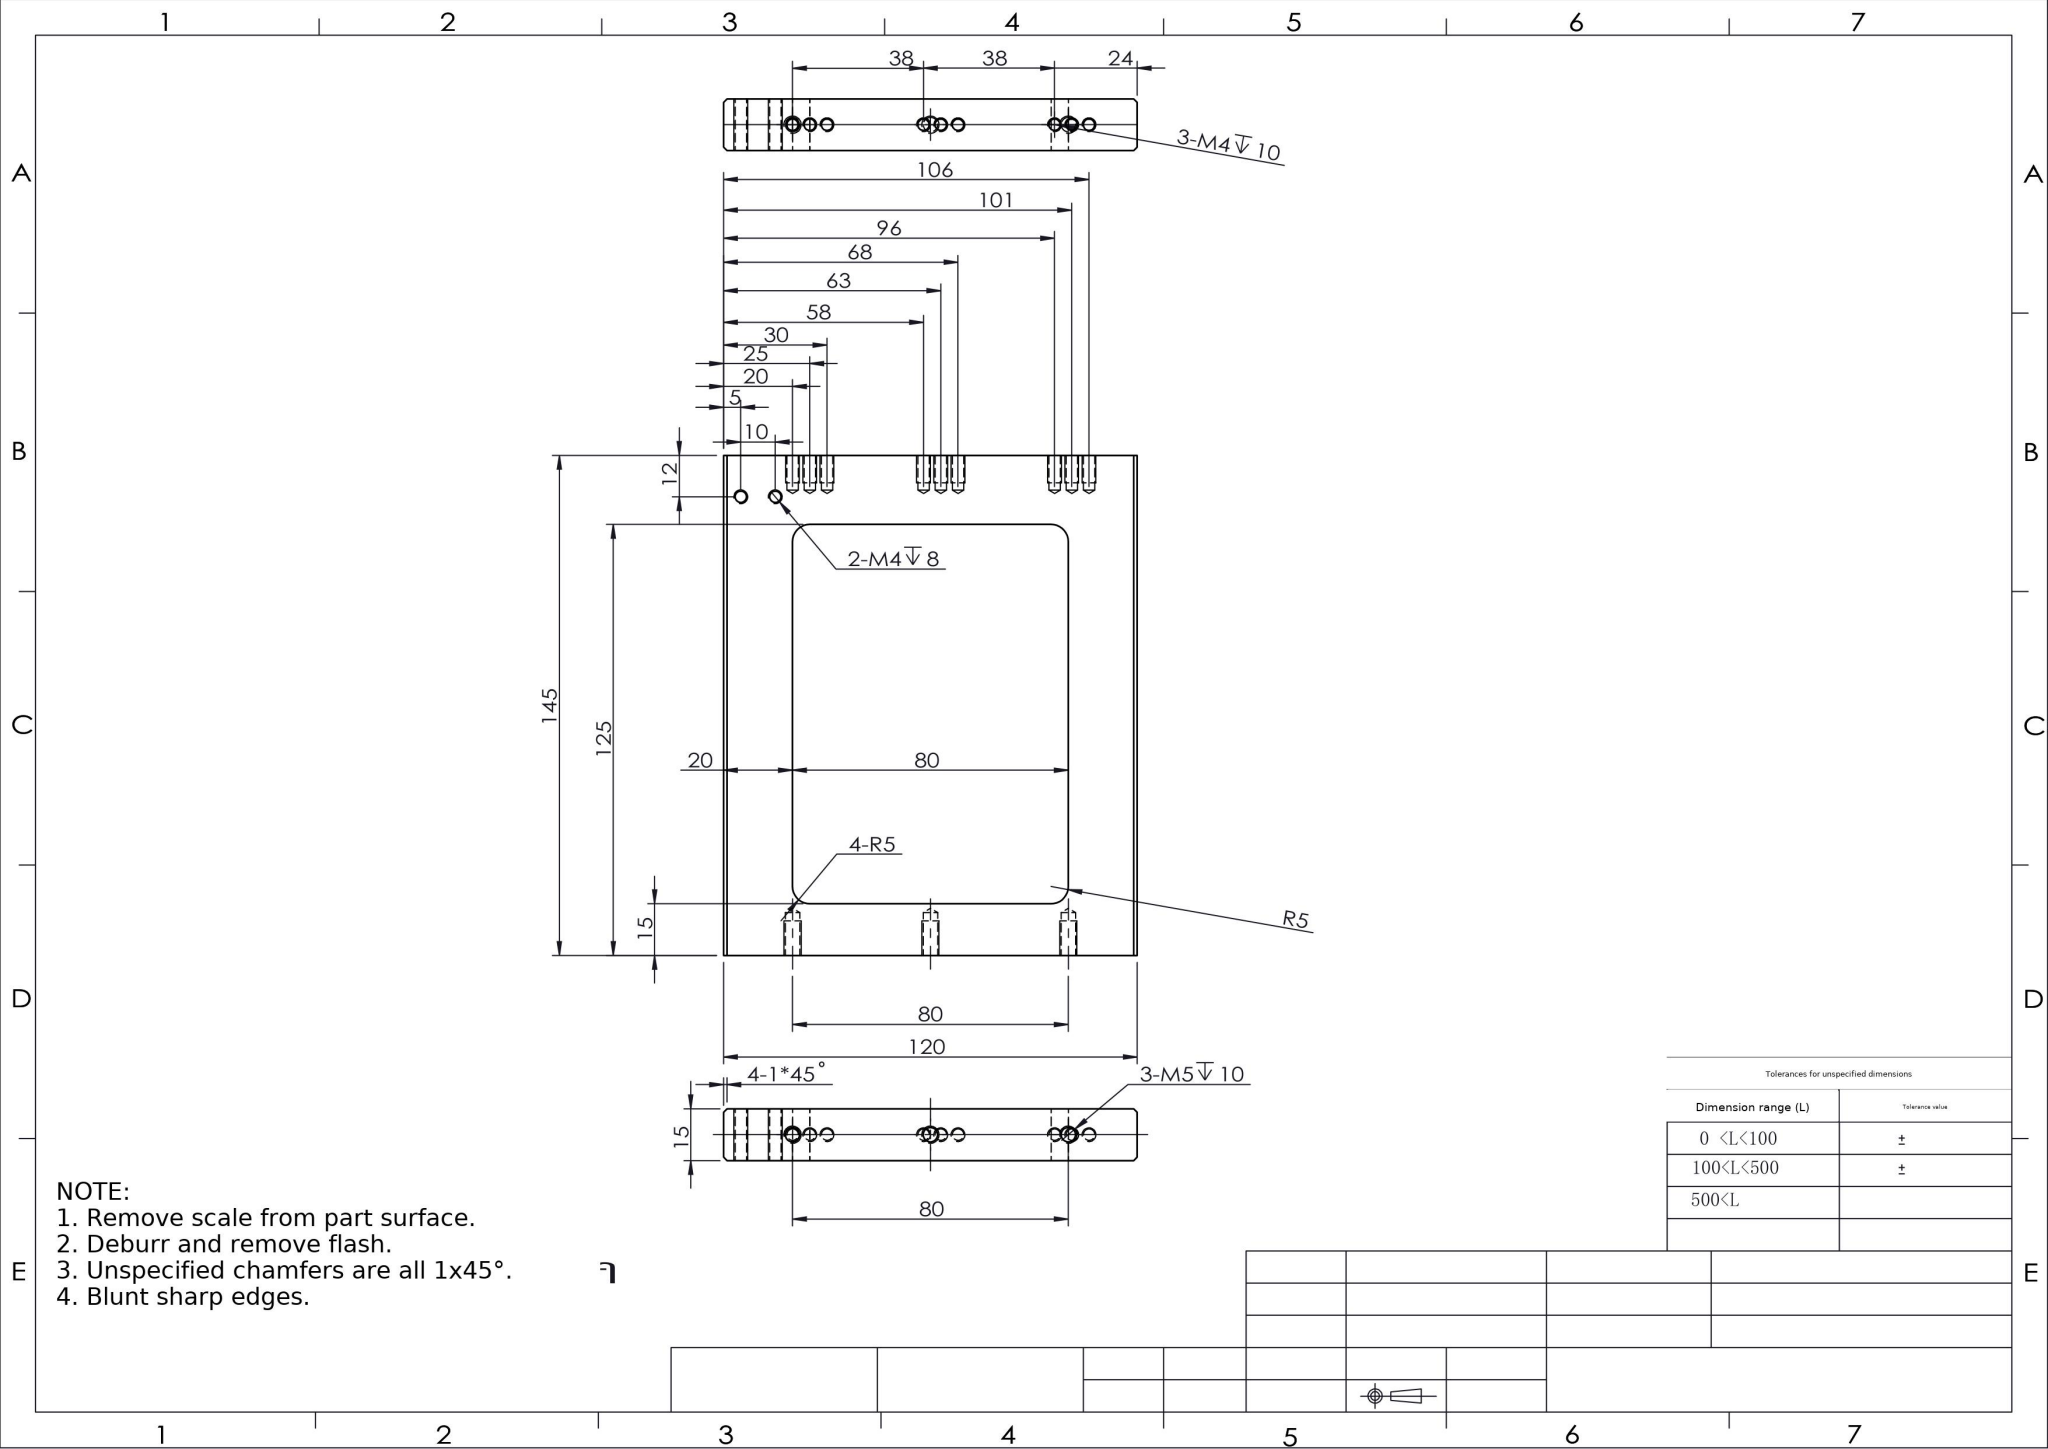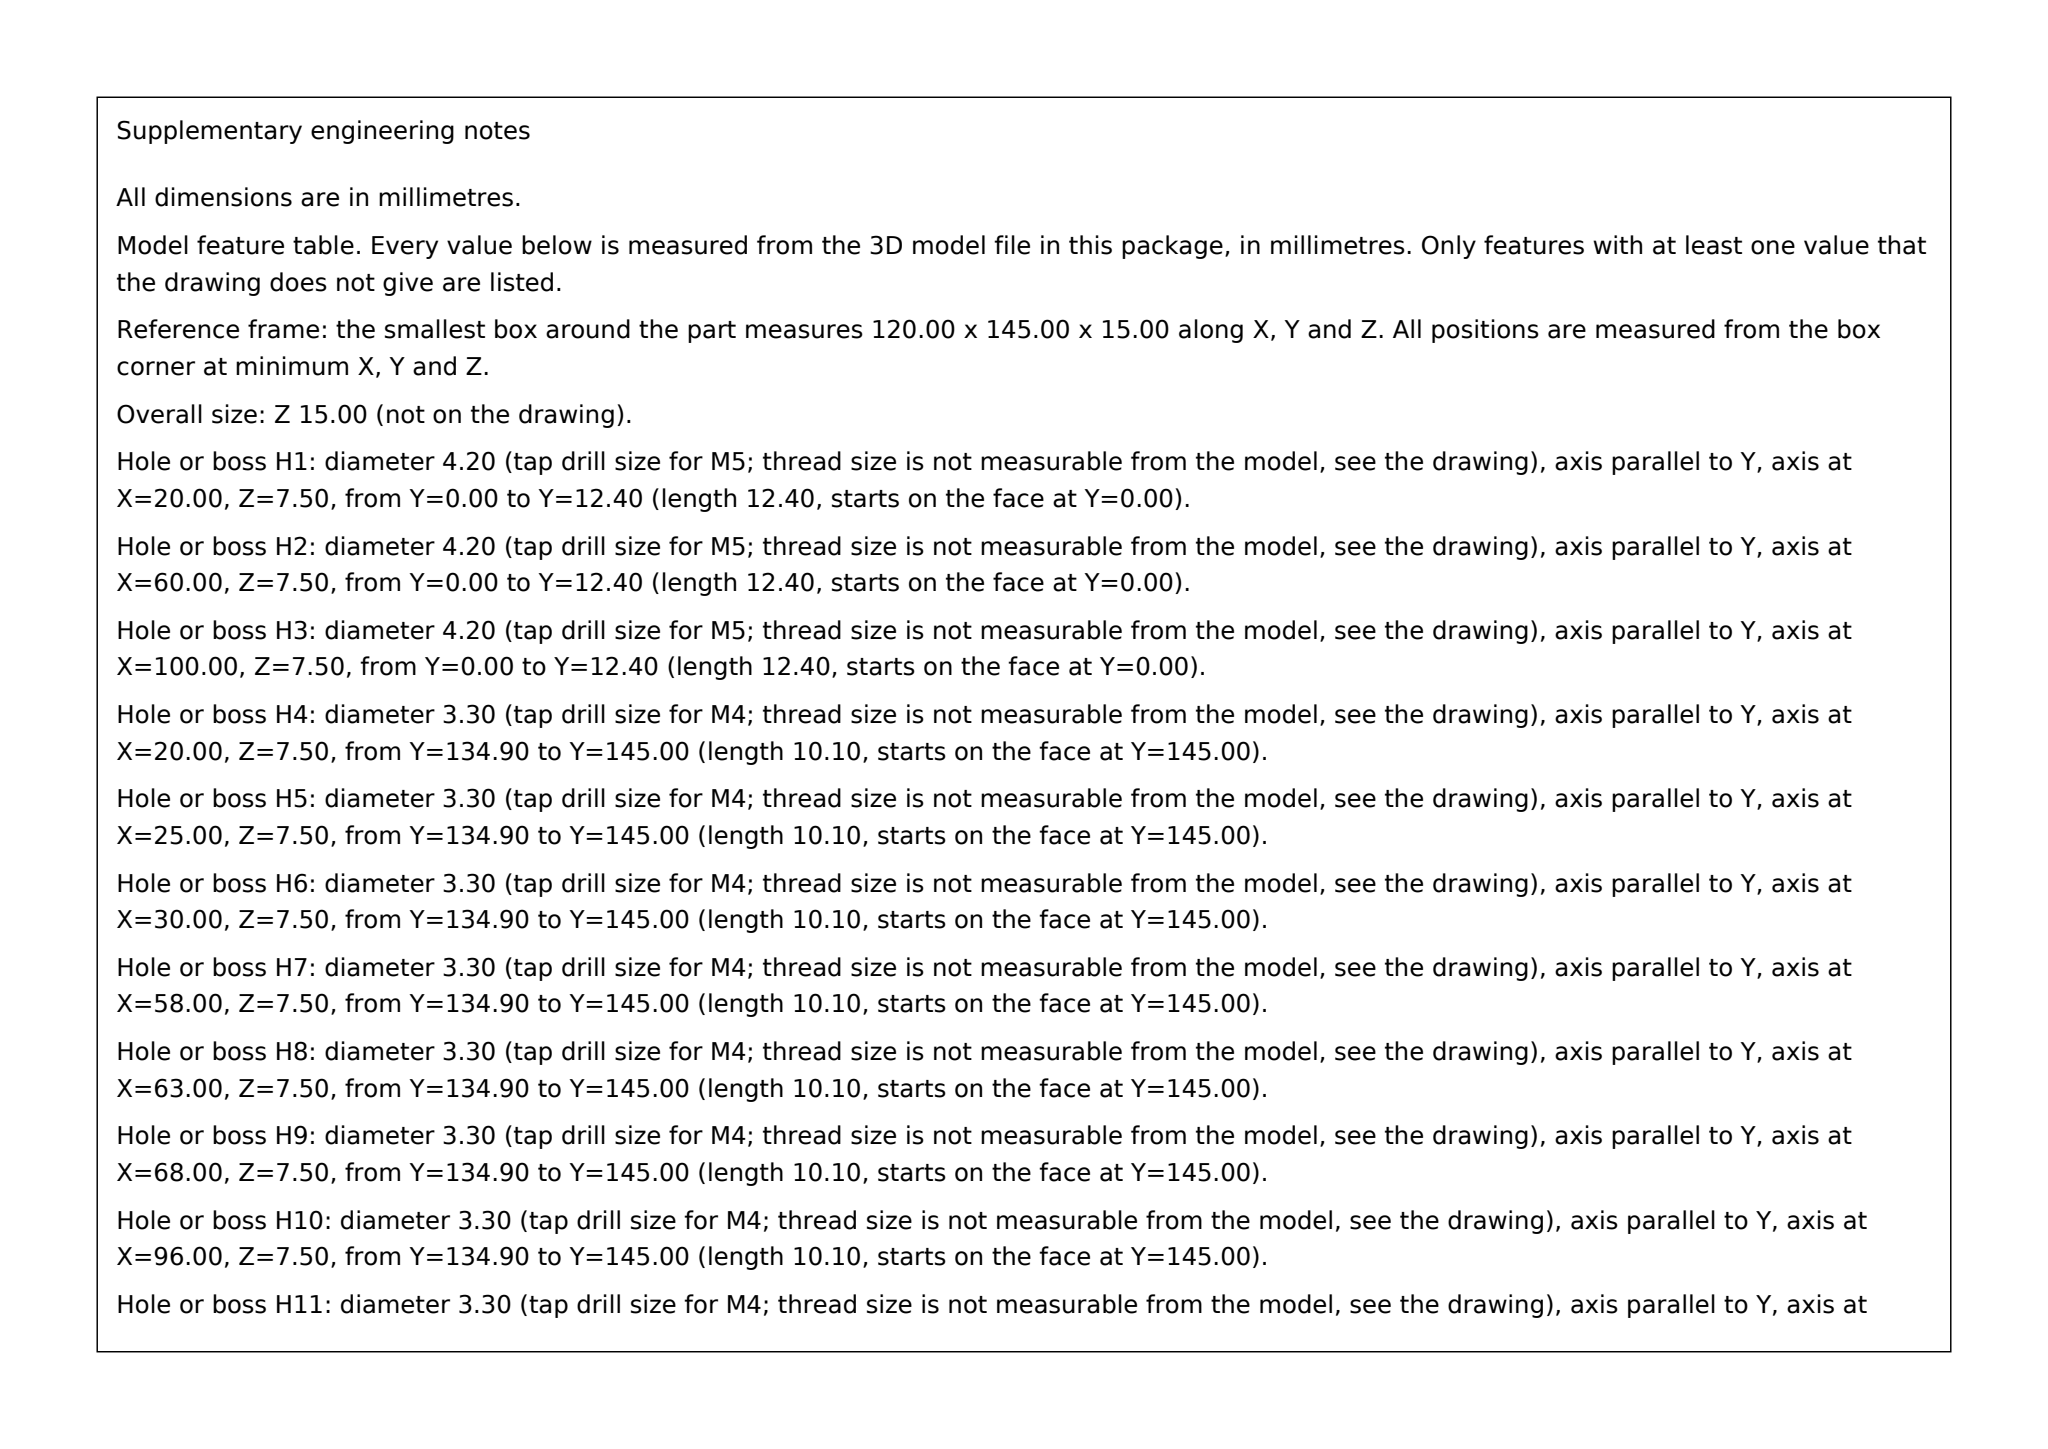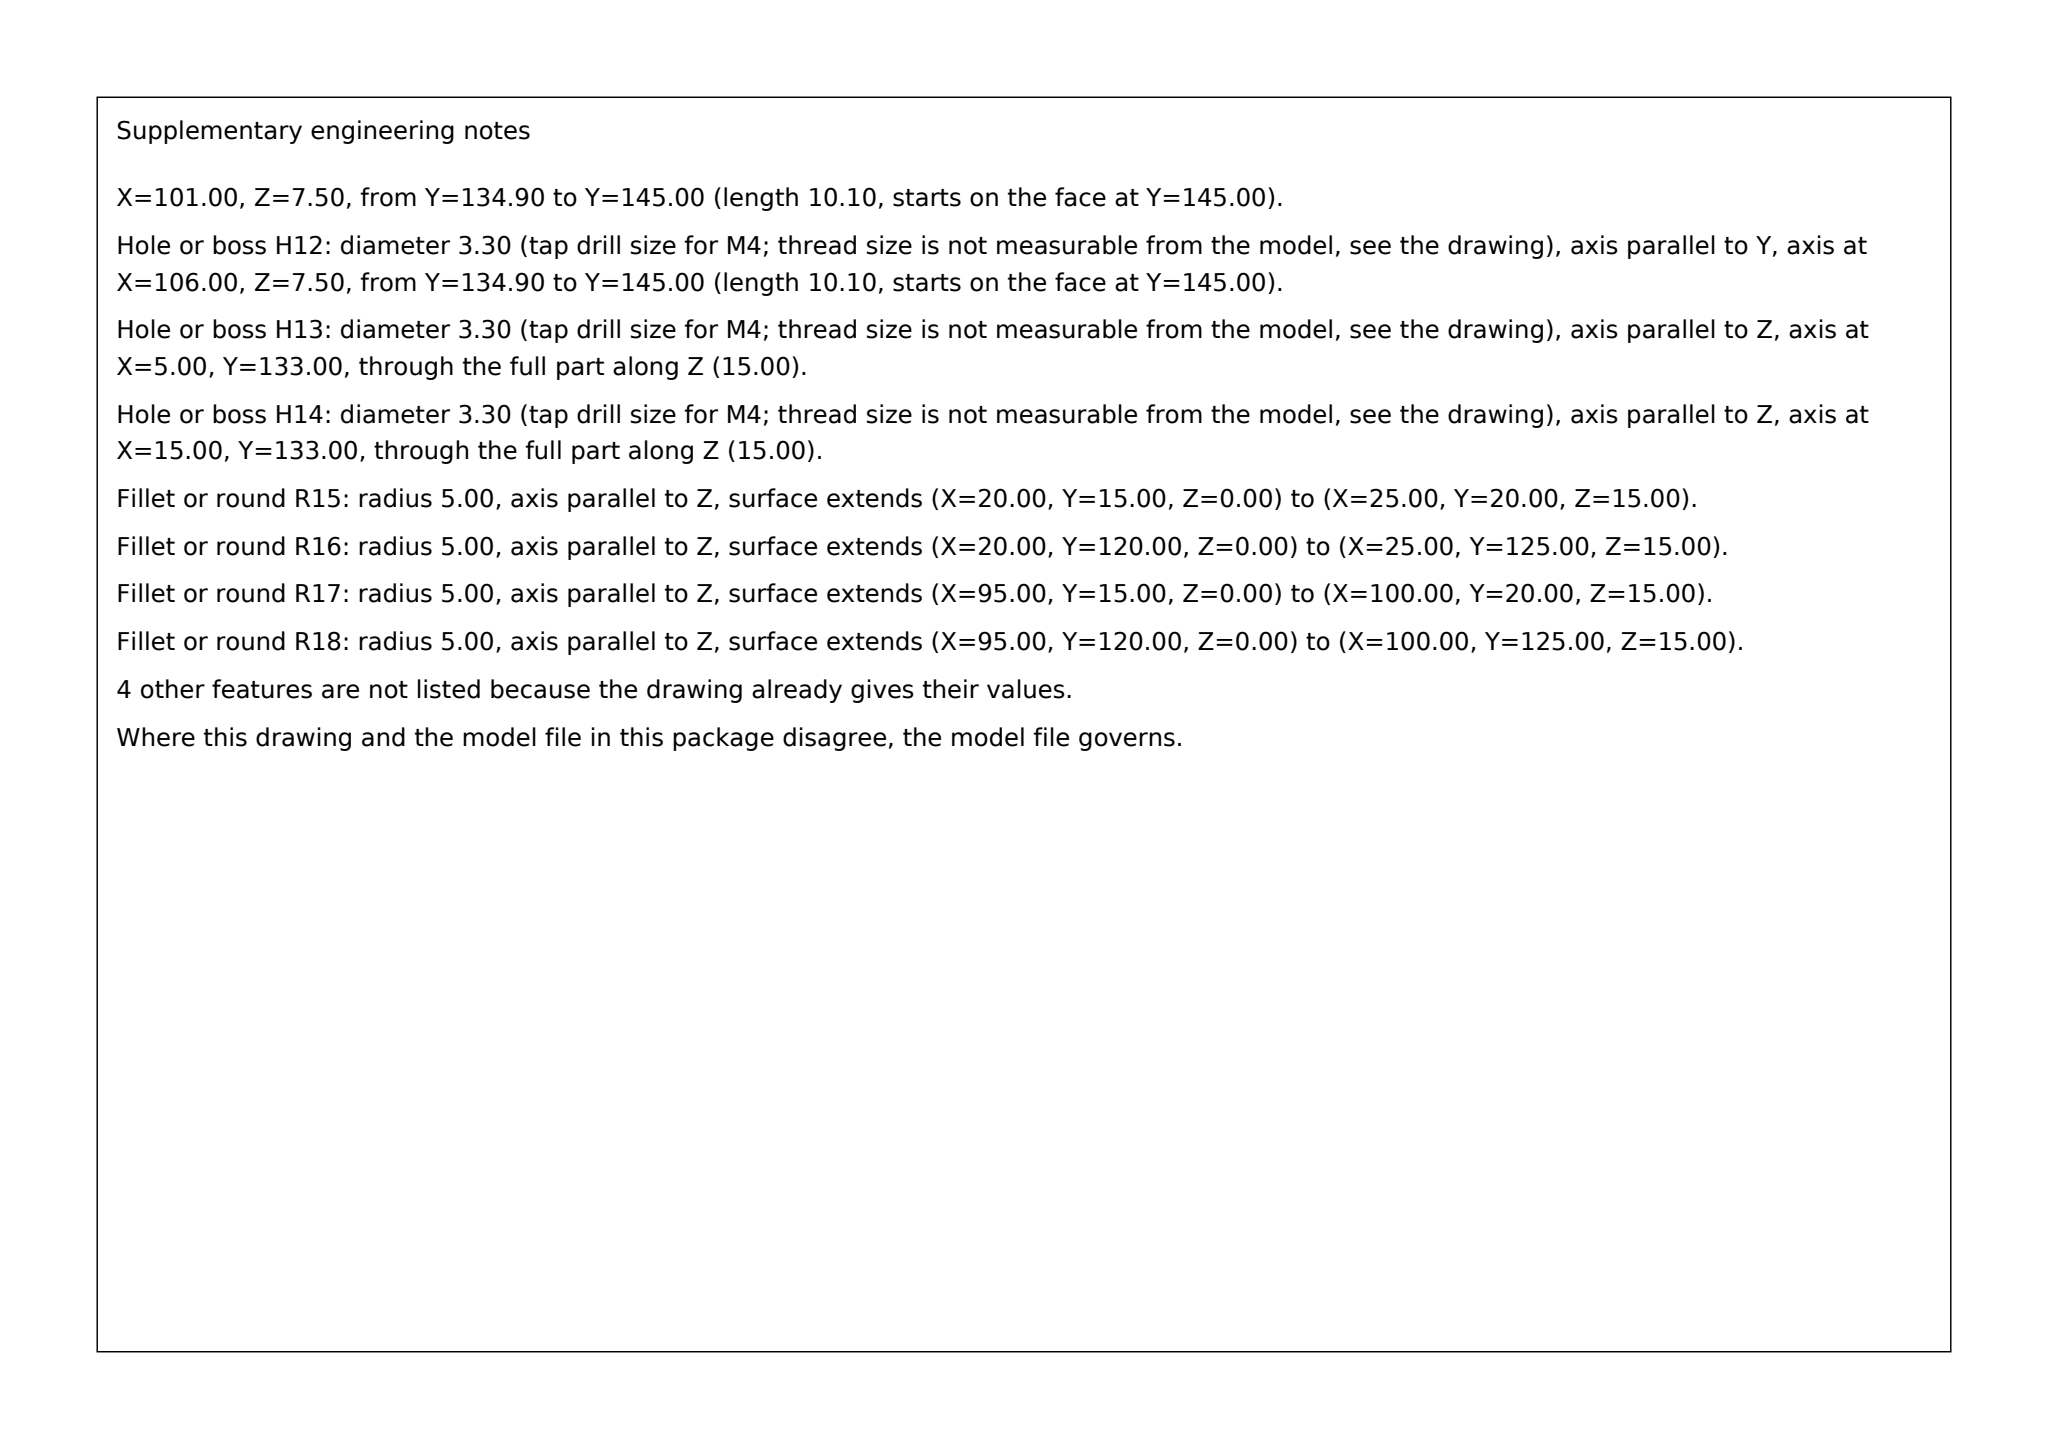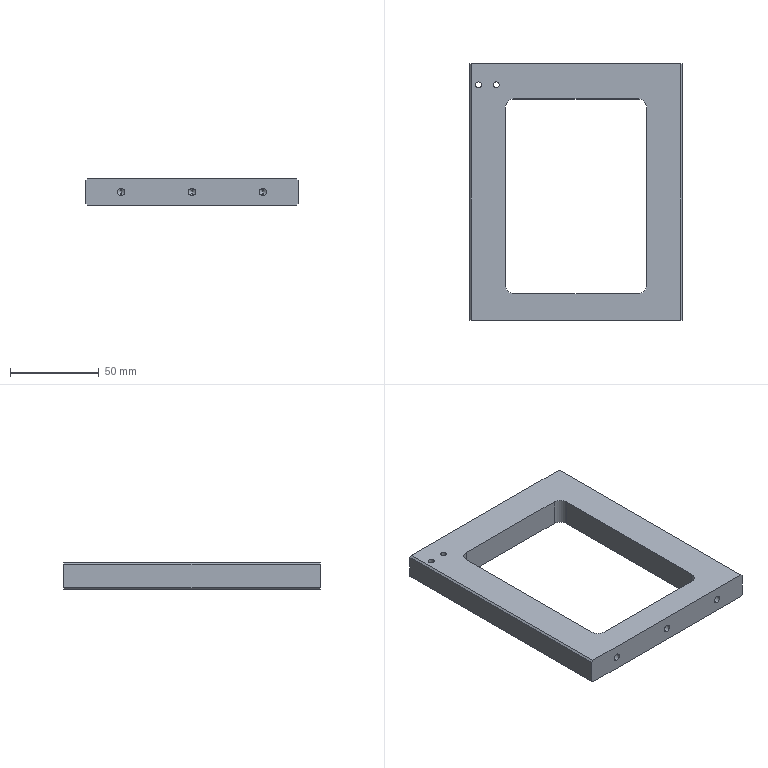Part | SolidWorks | mm | 1 solid | 70 faces | box 120 x 145 x 15 mm | volume 127440 mm3 | cylinder 32 | cone 24 | plane 14 | commonest cylinder face diameters 3.3 x22 4.2 x6 10 x4
build123d program:
from build123d import *

# Parameters (mm, degrees)
SKETCH1_W             = 120
SKETCH1_H             = 145
BOSS_EXTRUDE1_DEPTH   = 15
M5_TAPPED_HOLE1_D     = 4.2
M5_TAPPED_HOLE1_DEPTH = 12.4
M5_TAPPED_HOLE1_TIP   = 1.262
SKETCH7_W             = 80
SKETCH7_H             = 110
CUT_EXTRUDE1_DEPTH    = 189.812
FILLET1_R             = 5
CHAMFER1_SIZE         = 1
SKETCH8_R             = 1.65
CUT_EXTRUDE2_DEPTH    = 189.812
LPATTERN1_COUNT       = 3
LPATTERN1_PITCH       = 38
LPATTERN3_COUNT       = 3
LPATTERN3_PITCH       = 5


with BuildPart() as part:
    # Sketch1 → Boss-Extrude1 (new body)
    with BuildSketch(Plane.XY):
        with Locations((60, 72.5)):
            Rectangle(SKETCH1_W, SKETCH1_H)
    extrude(amount=BOSS_EXTRUDE1_DEPTH)

    # M5 Tapped Hole1
    with Locations(Plane(origin=(0, 0, 0), x_dir=(-1, 0, 0), z_dir=(0, -1, 0))):
        with Locations((-20, -7.5), (-60, -7.5), (-100, -7.5)):
            Hole(M5_TAPPED_HOLE1_D / 2, depth=M5_TAPPED_HOLE1_DEPTH)
            with Locations((0, 0, -(M5_TAPPED_HOLE1_DEPTH + M5_TAPPED_HOLE1_TIP / 2))):  # 118° drill point
                Cone(0, M5_TAPPED_HOLE1_D / 2, M5_TAPPED_HOLE1_TIP, mode=Mode.SUBTRACT)

    # Sketch7 → Cut-Extrude1 (cut, through all)
    with BuildSketch(Plane.XY.offset(15)):
        with Locations((60, 70)):
            Rectangle(SKETCH7_W, SKETCH7_H)
    extrude(amount=-CUT_EXTRUDE1_DEPTH, mode=Mode.SUBTRACT)

    # Fillet1
    fillet1_edges = [part.edges().sort_by_distance(p)[0] for p in [
        (20, 15, 7.5),
        (20, 125, 7.5),
        (100, 125, 7.5),
        (100, 15, 7.5),
    ]]
    fillet(fillet1_edges, radius=FILLET1_R)

    # Chamfer1
    chamfer1_edges = [part.edges().sort_by_distance(p)[0] for p in [
        (120, 72.5, 15),
        (0, 72.5, 15),
        (120, 72.5, 0),
        (0, 72.5, 0),
    ]]
    chamfer(chamfer1_edges, length=CHAMFER1_SIZE)

    # Sketch8 → Cut-Extrude2 (cut, through all)
    with BuildSketch(Plane(origin=(0, 0, 0), x_dir=(-1, 0, 0), z_dir=(0, 0, -1))):
        with Locations((-15, 133)):
            Circle(SKETCH8_R)
        with Locations((-5, 133)):
            Circle(SKETCH8_R)
    extrude(amount=-CUT_EXTRUDE2_DEPTH, mode=Mode.SUBTRACT)

    # Sketch4 → M4 Tapped Hole1 (revolve, cut)
    with BuildSketch(Plane(origin=(20, 145, 7.5), x_dir=(0, 0, 1), z_dir=(1, 0, 0))):
        Polygon((0, 0), (0, 11.091), (1.65, 10.1), (1.65, 0), align=None)
    m4_tapped_hole1 = revolve(axis=Axis((20, 151.35, 7.5), (0, -1, 0)), mode=Mode.SUBTRACT)

    # LPattern1: M4 Tapped Hole1 ×3
    with Locations(*[(i * LPATTERN1_PITCH, 0, 0) for i in range(1, LPATTERN1_COUNT)]):
        add(m4_tapped_hole1, mode=Mode.SUBTRACT)

    # LPattern3: M4 Tapped Hole1 ×3
    with Locations(*[(i * LPATTERN3_PITCH, 0, 0) for i in range(1, LPATTERN3_COUNT)]):
        add(m4_tapped_hole1, mode=Mode.SUBTRACT)

    # LPattern3 copy 1 sketch → LPattern3 copy 1 (revolve, cut)
    with BuildSketch(Plane(origin=(63, 145, 7.5), x_dir=(0, 0, 1), z_dir=(1, 0, 0))):
        Polygon((0, 0), (0, 11.091), (1.65, 10.1), (1.65, 0), align=None)
    revolve(axis=Axis((63, 151.35, 7.5), (0, -1, 0)), mode=Mode.SUBTRACT)

    # LPattern3 copy 2 sketch → LPattern3 copy 2 (revolve, cut)
    with BuildSketch(Plane(origin=(68, 145, 7.5), x_dir=(0, 0, 1), z_dir=(1, 0, 0))):
        Polygon((0, 0), (0, 11.091), (1.65, 10.1), (1.65, 0), align=None)
    revolve(axis=Axis((68, 151.35, 7.5), (0, -1, 0)), mode=Mode.SUBTRACT)

    # LPattern3 copy 3 sketch → LPattern3 copy 3 (revolve, cut)
    with BuildSketch(Plane(origin=(101, 145, 7.5), x_dir=(0, 0, 1), z_dir=(1, 0, 0))):
        Polygon((0, 0), (0, 11.091), (1.65, 10.1), (1.65, 0), align=None)
    revolve(axis=Axis((101, 151.35, 7.5), (0, -1, 0)), mode=Mode.SUBTRACT)

    # LPattern3 copy 4 sketch → LPattern3 copy 4 (revolve, cut)
    with BuildSketch(Plane(origin=(106, 145, 7.5), x_dir=(0, 0, 1), z_dir=(1, 0, 0))):
        Polygon((0, 0), (0, 11.091), (1.65, 10.1), (1.65, 0), align=None)
    revolve(axis=Axis((106, 151.35, 7.5), (0, -1, 0)), mode=Mode.SUBTRACT)


solid = part.part